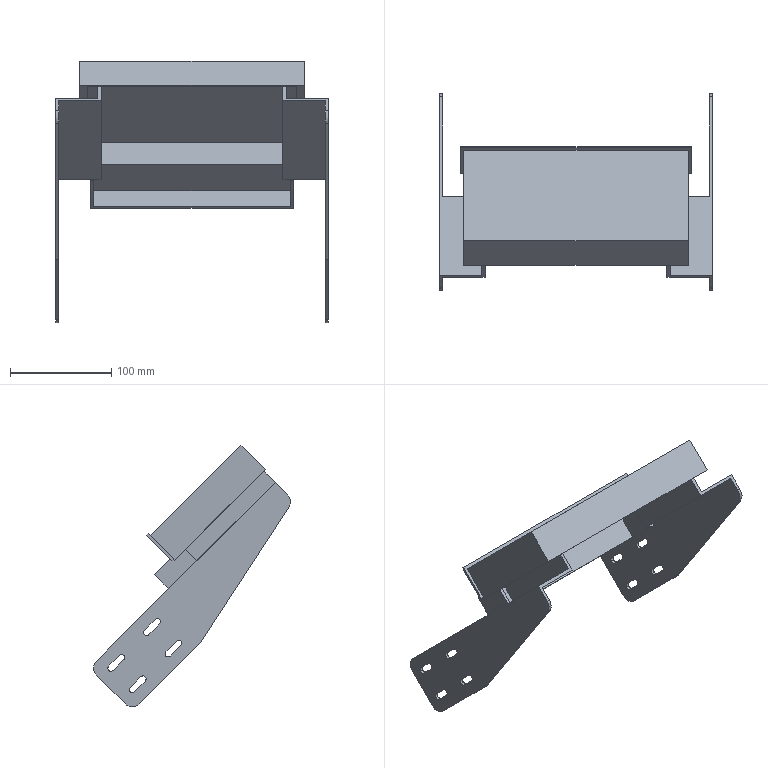Component | SolidWorks | Section5-1 | 2 solids | 120 faces | box 270 x 194.58 x 258.9 mm | volume 284650 mm3 | plane 90 | cylinder 30 | commonest cylinder face diameters 6 x24 20 x6
build123d program:
from build123d import *

# Parameters (mm, degrees)
EXTRUDE_THIN1_DEPTH      = 125
SKETCH2_W                = 222
SKETCH2_H                = 34
BOSS_EXTRUDE1_DEPTH      = 2
BOSS_EXTRUDE2_DEPTH      = 2
SKETCH4_W                = 3
SKETCH4_H                = 110
BOSS_EXTRUDE3_DEPTH      = 48
SKETCH5_W                = 45
SKETCH5_H                = 110
BOSS_EXTRUDE4_DEPTH      = 3
BOSS_EXTRUDE5_DEPTH      = 3
BOSS_EXTRUDE6_DEPTH      = 3
BOSS_EXTRUDE7_DEPTH      = 22
BOSS_EXTRUDE7_DEPTH_BACK = 17
SKETCH9_W                = 200
SKETCH9_H                = 25
SHELL1_T                 = -3
EXTRUDE_THIN2_START      = -31
SKETCH10_W               = 194
SKETCH10_H               = 2
EXTRUDE_THIN2_DEPTH      = 28
FILLET1_R                = 10
CUT_EXTRUDE1_DEPTH       = 313.357
LPATTERN1_COUNT          = 2
LPATTERN1_PITCH          = 50
LPATTERN1_COUNT_DIR2     = 2
LPATTERN1_PITCH_DIR2     = 30


with BuildPart() as part:
    # Sketch1 → Extrude-Thin1 (new body)
    with BuildSketch(Plane.XY):
        Polygon((-53.736, -13.736), (-61.736, -13.736), (-61.736, 20.264), (160.264, 20.264), (160.264, -13.736), (152.264, -13.736), (152.264, -11.736), (158.264, -11.736), (158.264, 18.264), (-59.736, 18.264), (-59.736, -11.736), (-53.736, -11.736), align=None)
    extrude(amount=EXTRUDE_THIN1_DEPTH)



with BuildPart() as body_2:
    # Sketch2 → Boss-Extrude1 (new body)
    with BuildSketch(Plane.XY.offset(125)):
        with Locations((49.264, 3.264)):
            Rectangle(SKETCH2_W, SKETCH2_H)
    extrude(amount=BOSS_EXTRUDE1_DEPTH)


with BuildPart() as body_3:
    # Sketch3 → Boss-Extrude2 (new body)
    with BuildSketch(Plane(origin=(0, 0, 0), x_dir=(-1, 0, 0), z_dir=(0, 0, -1))):
        Polygon((-151.264, -11.736), (-163.264, -11.736), (-163.264, 23.264), (64.736, 23.264), (64.736, -11.736), (52.736, -11.736), (52.736, -9.736), (12.736, -9.736), (12.736, 0.2637), (2.736, 10.264), (-101.264, 10.264), (-111.264, 0.2637), (-111.264, -9.736), (-151.264, -9.736), align=None)
    extrude(amount=BOSS_EXTRUDE2_DEPTH)


with BuildPart() as part_1:
    add(part.part)

    add(body_2.part)  # Boss-Extrude3 merges body 2
    # Sketch4 → Boss-Extrude3 (add)
    with BuildSketch(Plane(origin=(0, 18.264, 0), x_dir=(-1, 0, 0), z_dir=(0, -1, 0))):
        with Locations((42.236, -70)):
            Rectangle(SKETCH4_W, SKETCH4_H)
        with Locations((-140.764, -70)):
            Rectangle(SKETCH4_W, SKETCH4_H)
    extrude(amount=BOSS_EXTRUDE3_DEPTH)

    # Sketch5 → Boss-Extrude4 (add)
    with BuildSketch(Plane.XZ.offset(29.736)):
        with Locations((-63.236, 70)):
            Rectangle(SKETCH5_W, SKETCH5_H)
        with Locations((161.764, 70)):
            Rectangle(SKETCH5_W, SKETCH5_H)
    extrude(amount=BOSS_EXTRUDE4_DEPTH)

    # Sketch6 → Boss-Extrude5 (add)
    with BuildSketch(Plane(origin=(184.264, 0, 0), x_dir=(0, 0, -1), z_dir=(1, 0, 0))):
        Polygon((-125, -29.736), (-125, -54.736), (40.455, -89.736), (135, -89.736), (135, -29.736), align=None)
    extrude(amount=-BOSS_EXTRUDE5_DEPTH)

    # Sketch7 → Boss-Extrude6 (add)
    with BuildSketch(Plane.ZY.offset(85.736)):
        Polygon((125, -29.736), (125, -54.736), (-40.455, -89.736), (-135, -89.736), (-135, -29.736), align=None)
    extrude(amount=-BOSS_EXTRUDE6_DEPTH)



with BuildPart() as body_3_2:
    # Sketch9 → Boss-Extrude7 (new, two sides: drawn at the far end of the back side and taken through both)
    with BuildSketch(Plane(origin=(0, 0, -2), x_dir=(-1, 0, 0), z_dir=(0, 0, -1)).offset(-BOSS_EXTRUDE7_DEPTH_BACK)):
        with Locations((-49.264, -22.236)):
            Rectangle(SKETCH9_W, SKETCH9_H)
    extrude(amount=BOSS_EXTRUDE7_DEPTH + BOSS_EXTRUDE7_DEPTH_BACK)

    # Shell1
    shell1_openings = [body_3_2.faces().sort_by_distance(p)[0] for p in [
        (49.264, -22.236, 15),
        (49.264, -34.736, -4.5),
    ]]
    offset(amount=SHELL1_T, openings=shell1_openings, kind=Kind.INTERSECTION)


with BuildPart() as part_2:
    add(part_1.part)

    add(body_3_2.part)  # Extrude-Thin2 merges body 3 2
    # Sketch10 → Extrude-Thin2 (add)
    with BuildSketch(Plane.XZ.offset(12.736).offset(EXTRUDE_THIN2_START)):
        with Locations((49.264, 14)):
            Rectangle(SKETCH10_W, SKETCH10_H)
    extrude(amount=EXTRUDE_THIN2_DEPTH)

    # Fillet1
    fillet1_edges = [part_2.edges().sort_by_distance(p)[0] for p in [
        (182.764, -29.736, -135),
        (182.764, -89.736, -135),
        (182.764, -54.736, 125),
        (-84.236, -29.736, -135),
        (-84.236, -54.736, 125),
        (-84.236, -89.736, -135),
    ]]
    fillet(fillet1_edges, radius=FILLET1_R)

    # Sketch11 → Cut-Extrude1 (cut, symmetric)
    with BuildSketch(Plane(origin=(-82.736, 0, 0), x_dir=(0, 0, -1), z_dir=(1, 0, 0))):
        with BuildLine():
            Line((105, -41.736), (120, -41.736))
            ThreePointArc((120, -41.736), (123, -44.736), (120, -47.736))
            Line((120, -47.736), (105, -47.736))
            ThreePointArc((105, -47.736), (102, -44.736), (105, -41.736))
        make_face()
    cut_extrude1 = extrude(amount=CUT_EXTRUDE1_DEPTH, both=True, mode=Mode.SUBTRACT)

    # LPattern1: Cut-Extrude1 2 × 2
    with Locations(*[(0, -j * LPATTERN1_PITCH_DIR2, i * LPATTERN1_PITCH) for i in range(LPATTERN1_COUNT) for j in range(LPATTERN1_COUNT_DIR2) if (i, j) != (0, 0)]):
        add(cut_extrude1, mode=Mode.SUBTRACT)


solid = Compound([body_3.part, part_2.part])

# Placed as in the assembly
solid = solid.moved(Location((69.561, -392.743, 164.064), (45, 0, 0)))